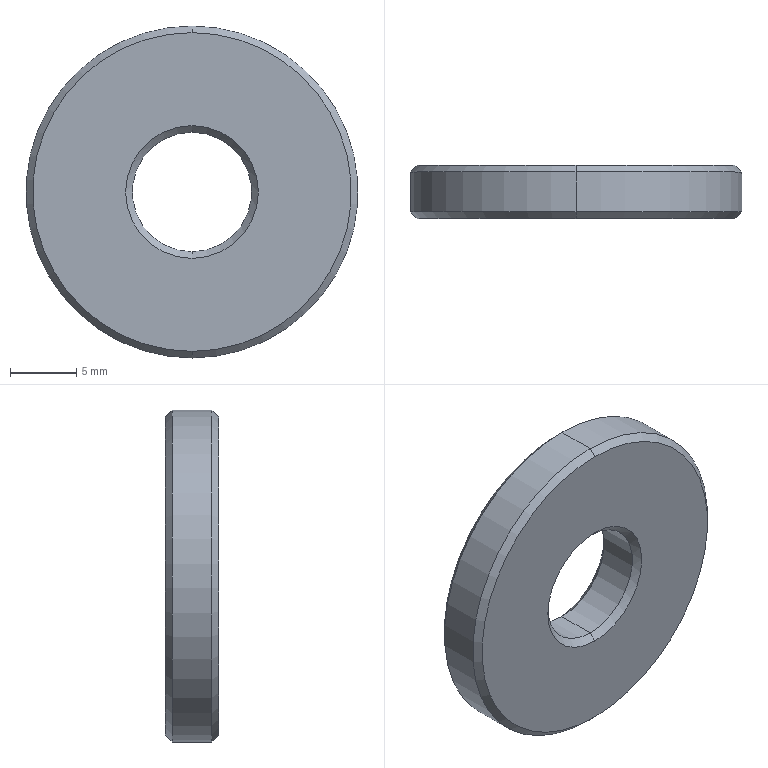Component | SolidWorks | Yk1.5.5EndCap-4 | 1 solid | 14 faces | box 25 x 4 x 25 mm | volume 1682 mm3 | cone 8 | cylinder 4 | plane 2 | commonest cylinder face diameters 9 x2 25 x2 | material 45
build123d program:
from build123d import *

# Parameters (mm, degrees)
SKETCH1_R           = 12.5
SKETCH1_R_2         = 4.5
BOSS_EXTRUDE1_DEPTH = 4
CHAMFER1_SIZE       = 0.5


with BuildPart() as part:
    # Sketch1 → Boss-Extrude1 (new body)
    with BuildSketch(Plane(origin=(0, 0, 0), x_dir=(1, 0, 0), z_dir=(0, 1, 0))):
        with Locations(Location((0, 0, 0), (0, 0, 270))):
            Circle(SKETCH1_R)
        with Locations(Location((0, 0, 0), (0, 0, 270))):
            Circle(SKETCH1_R_2, mode=Mode.SUBTRACT)
    extrude(amount=BOSS_EXTRUDE1_DEPTH)

    # Chamfer1
    chamfer1_edges = [part.edges().sort_by_distance(p)[0] for p in [
        (0, 0, -12.5),
        (0, 4, -12.5),
        (0, 0, -4.5),
        (0, 4, -4.5),
    ]]
    chamfer(chamfer1_edges, length=CHAMFER1_SIZE)


solid = part.part

# Placed as in the assembly
solid = solid.moved(Location((-41.072, -44, 23.739), (0, 0, 0)))
STEP:
#1=COLOUR_RGB('',0.7922,0.8196,0.9333);
#2=FILL_AREA_STYLE_COLOUR('',#1);
#3=FILL_AREA_STYLE('',(#2));
#4=SURFACE_STYLE_FILL_AREA(#3);
#5=SURFACE_SIDE_STYLE('',(#4));
#6=SURFACE_STYLE_USAGE(.BOTH.,#5);
#7=PRESENTATION_STYLE_ASSIGNMENT((#6));
#8=CARTESIAN_POINT('',(-1.617,-1.732,0.4621));
#9=VERTEX_POINT('',#8);
#10=CARTESIAN_POINT('',(-1.617,-1.732,1.407));
#11=VERTEX_POINT('',#10);
#12=CARTESIAN_POINT('',(-1.617,-1.732,0.9346));
#13=DIRECTION('',(0.,-1.,0.));
#14=DIRECTION('',(0.,0.,1.));
#15=AXIS2_PLACEMENT_3D('',#12,#13,#14);
#16=CIRCLE('',#15,0.4724);
#17=EDGE_CURVE('',#9,#11,#16,.T.);
#18=ORIENTED_EDGE('',*,*,#17,.F.);
#19=CARTESIAN_POINT('',(-1.617,-1.713,0.4425));
#20=VERTEX_POINT('',#19);
#21=CARTESIAN_POINT('',(-1.617,-1.713,0.4425));
#22=DIRECTION('',(0.,0.7071,-0.7071));
#23=VECTOR('',#22,39.37);
#24=LINE('',#21,#23);
#25=EDGE_CURVE('',#9,#20,#24,.T.);
#26=ORIENTED_EDGE('',*,*,#25,.T.);
#27=CARTESIAN_POINT('',(-1.617,-1.713,1.427));
#28=VERTEX_POINT('',#27);
#29=CARTESIAN_POINT('',(-1.617,-1.713,0.9346));
#30=DIRECTION('',(0.,1.,0.));
#31=DIRECTION('',(0.,0.,1.));
#32=AXIS2_PLACEMENT_3D('',#29,#30,#31);
#33=CIRCLE('',#32,0.4921);
#34=EDGE_CURVE('',#28,#20,#33,.T.);
#35=ORIENTED_EDGE('',*,*,#34,.F.);
#36=CARTESIAN_POINT('',(-1.617,-1.713,1.427));
#37=DIRECTION('',(0.,0.7071,0.7071));
#38=VECTOR('',#37,39.37);
#39=LINE('',#36,#38);
#40=EDGE_CURVE('',#11,#28,#39,.T.);
#41=ORIENTED_EDGE('',*,*,#40,.F.);
#42=EDGE_LOOP('',(#18,#26,#35,#41));
#43=FACE_OUTER_BOUND('',#42,.T.);
#44=CARTESIAN_POINT('',(-1.617,-1.713,0.9346));
#45=DIRECTION('',(0.,1.,0.));
#46=DIRECTION('',(0.,0.,1.));
#47=AXIS2_PLACEMENT_3D('',#44,#45,#46);
#48=CONICAL_SURFACE('',#47,0.4921,0.7854);
#49=ADVANCED_FACE('',(#43),#48,.T.);
#50=CARTESIAN_POINT('',(-1.617,-1.713,1.112));
#51=VERTEX_POINT('',#50);
#52=CARTESIAN_POINT('',(-1.617,-1.713,0.7574));
#53=VERTEX_POINT('',#52);
#54=CARTESIAN_POINT('',(-1.617,-1.713,0.9346));
#55=DIRECTION('',(0.,-1.,0.));
#56=DIRECTION('',(0.,0.,1.));
#57=AXIS2_PLACEMENT_3D('',#54,#55,#56);
#58=CIRCLE('',#57,0.1772);
#59=EDGE_CURVE('',#51,#53,#58,.T.);
#60=ORIENTED_EDGE('',*,*,#59,.F.);
#61=CARTESIAN_POINT('',(-1.617,-1.732,1.131));
#62=VERTEX_POINT('',#61);
#63=CARTESIAN_POINT('',(-1.617,-1.732,1.131));
#64=DIRECTION('',(0.,-0.7071,0.7071));
#65=VECTOR('',#64,39.37);
#66=LINE('',#63,#65);
#67=EDGE_CURVE('',#51,#62,#66,.T.);
#68=ORIENTED_EDGE('',*,*,#67,.T.);
#69=CARTESIAN_POINT('',(-1.617,-1.732,0.7377));
#70=VERTEX_POINT('',#69);
#71=CARTESIAN_POINT('',(-1.617,-1.732,0.9346));
#72=DIRECTION('',(0.,1.,0.));
#73=DIRECTION('',(0.,0.,1.));
#74=AXIS2_PLACEMENT_3D('',#71,#72,#73);
#75=CIRCLE('',#74,0.1969);
#76=EDGE_CURVE('',#70,#62,#75,.T.);
#77=ORIENTED_EDGE('',*,*,#76,.F.);
#78=CARTESIAN_POINT('',(-1.617,-1.732,0.7377));
#79=DIRECTION('',(0.,-0.7071,-0.7071));
#80=VECTOR('',#79,39.37);
#81=LINE('',#78,#80);
#82=EDGE_CURVE('',#53,#70,#81,.T.);
#83=ORIENTED_EDGE('',*,*,#82,.F.);
#84=EDGE_LOOP('',(#60,#68,#77,#83));
#85=FACE_OUTER_BOUND('',#84,.T.);
#86=CARTESIAN_POINT('',(-1.617,-1.732,0.9346));
#87=DIRECTION('',(0.,-1.,0.));
#88=DIRECTION('',(0.,0.,-1.));
#89=AXIS2_PLACEMENT_3D('',#86,#87,#88);
#90=CONICAL_SURFACE('',#89,0.1969,0.7854);
#91=ADVANCED_FACE('',(#85),#90,.F.);
#92=CARTESIAN_POINT('',(-1.617,-1.575,1.407));
#93=VERTEX_POINT('',#92);
#94=CARTESIAN_POINT('',(-1.617,-1.575,0.4621));
#95=VERTEX_POINT('',#94);
#96=CARTESIAN_POINT('',(-1.617,-1.575,0.9346));
#97=DIRECTION('',(0.,1.,0.));
#98=DIRECTION('',(0.,0.,1.));
#99=AXIS2_PLACEMENT_3D('',#96,#97,#98);
#100=CIRCLE('',#99,0.4724);
#101=EDGE_CURVE('',#93,#95,#100,.T.);
#102=ORIENTED_EDGE('',*,*,#101,.F.);
#103=CARTESIAN_POINT('',(-1.617,-1.594,1.427));
#104=VERTEX_POINT('',#103);
#105=CARTESIAN_POINT('',(-1.617,-1.575,1.407));
#106=DIRECTION('',(0.,-0.7071,0.7071));
#107=VECTOR('',#106,39.37);
#108=LINE('',#105,#107);
#109=EDGE_CURVE('',#93,#104,#108,.T.);
#110=ORIENTED_EDGE('',*,*,#109,.T.);
#111=CARTESIAN_POINT('',(-1.617,-1.594,0.4425));
#112=VERTEX_POINT('',#111);
#113=CARTESIAN_POINT('',(-1.617,-1.594,0.9346));
#114=DIRECTION('',(0.,-1.,0.));
#115=DIRECTION('',(0.,0.,1.));
#116=AXIS2_PLACEMENT_3D('',#113,#114,#115);
#117=CIRCLE('',#116,0.4921);
#118=EDGE_CURVE('',#112,#104,#117,.T.);
#119=ORIENTED_EDGE('',*,*,#118,.F.);
#120=CARTESIAN_POINT('',(-1.617,-1.575,0.4621));
#121=DIRECTION('',(0.,-0.7071,-0.7071));
#122=VECTOR('',#121,39.37);
#123=LINE('',#120,#122);
#124=EDGE_CURVE('',#95,#112,#123,.T.);
#125=ORIENTED_EDGE('',*,*,#124,.F.);
#126=EDGE_LOOP('',(#102,#110,#119,#125));
#127=FACE_OUTER_BOUND('',#126,.T.);
#128=CARTESIAN_POINT('',(-1.617,-1.575,0.9346));
#129=DIRECTION('',(0.,-1.,0.));
#130=DIRECTION('',(0.,0.,-1.));
#131=AXIS2_PLACEMENT_3D('',#128,#129,#130);
#132=CONICAL_SURFACE('',#131,0.4724,0.7854);
#133=ADVANCED_FACE('',(#127),#132,.T.);
#134=CARTESIAN_POINT('',(-1.617,-1.594,0.7574));
#135=VERTEX_POINT('',#134);
#136=CARTESIAN_POINT('',(-1.617,-1.594,1.112));
#137=VERTEX_POINT('',#136);
#138=CARTESIAN_POINT('',(-1.617,-1.594,0.9346));
#139=DIRECTION('',(0.,1.,0.));
#140=DIRECTION('',(0.,0.,1.));
#141=AXIS2_PLACEMENT_3D('',#138,#139,#140);
#142=CIRCLE('',#141,0.1772);
#143=EDGE_CURVE('',#135,#137,#142,.T.);
#144=ORIENTED_EDGE('',*,*,#143,.F.);
#145=CARTESIAN_POINT('',(-1.617,-1.575,0.7377));
#146=VERTEX_POINT('',#145);
#147=CARTESIAN_POINT('',(-1.617,-1.594,0.7574));
#148=DIRECTION('',(0.,0.7071,-0.7071));
#149=VECTOR('',#148,39.37);
#150=LINE('',#147,#149);
#151=EDGE_CURVE('',#135,#146,#150,.T.);
#152=ORIENTED_EDGE('',*,*,#151,.T.);
#153=CARTESIAN_POINT('',(-1.617,-1.575,1.131));
#154=VERTEX_POINT('',#153);
#155=CARTESIAN_POINT('',(-1.617,-1.575,0.9346));
#156=DIRECTION('',(0.,-1.,0.));
#157=DIRECTION('',(0.,0.,1.));
#158=AXIS2_PLACEMENT_3D('',#155,#156,#157);
#159=CIRCLE('',#158,0.1969);
#160=EDGE_CURVE('',#154,#146,#159,.T.);
#161=ORIENTED_EDGE('',*,*,#160,.F.);
#162=CARTESIAN_POINT('',(-1.617,-1.594,1.112));
#163=DIRECTION('',(0.,0.7071,0.7071));
#164=VECTOR('',#163,39.37);
#165=LINE('',#162,#164);
#166=EDGE_CURVE('',#137,#154,#165,.T.);
#167=ORIENTED_EDGE('',*,*,#166,.F.);
#168=EDGE_LOOP('',(#144,#152,#161,#167));
#169=FACE_OUTER_BOUND('',#168,.T.);
#170=CARTESIAN_POINT('',(-1.617,-1.594,0.9346));
#171=DIRECTION('',(0.,1.,0.));
#172=DIRECTION('',(0.,0.,1.));
#173=AXIS2_PLACEMENT_3D('',#170,#171,#172);
#174=CONICAL_SURFACE('',#173,0.1772,0.7854);
#175=ADVANCED_FACE('',(#169),#174,.F.);
#176=ORIENTED_EDGE('',*,*,#143,.T.);
#177=CARTESIAN_POINT('',(-1.617,-1.575,1.112));
#178=DIRECTION('',(0.,-1.,0.));
#179=VECTOR('',#178,39.37);
#180=LINE('',#177,#179);
#181=EDGE_CURVE('',#137,#51,#180,.T.);
#182=ORIENTED_EDGE('',*,*,#181,.T.);
#183=ORIENTED_EDGE('',*,*,#59,.T.);
#184=CARTESIAN_POINT('',(-1.617,-1.575,0.7574));
#185=DIRECTION('',(0.,-1.,0.));
#186=VECTOR('',#185,39.37);
#187=LINE('',#184,#186);
#188=EDGE_CURVE('',#135,#53,#187,.T.);
#189=ORIENTED_EDGE('',*,*,#188,.F.);
#190=EDGE_LOOP('',(#176,#182,#183,#189));
#191=FACE_OUTER_BOUND('',#190,.T.);
#192=CARTESIAN_POINT('',(-1.617,-1.575,0.9346));
#193=DIRECTION('',(0.,-1.,0.));
#194=DIRECTION('',(0.,0.,-1.));
#195=AXIS2_PLACEMENT_3D('',#192,#193,#194);
#196=CYLINDRICAL_SURFACE('',#195,0.1772);
#197=ADVANCED_FACE('',(#191),#196,.F.);
#198=ORIENTED_EDGE('',*,*,#118,.T.);
#199=CARTESIAN_POINT('',(-1.617,-1.575,1.427));
#200=DIRECTION('',(0.,-1.,0.));
#201=VECTOR('',#200,39.37);
#202=LINE('',#199,#201);
#203=EDGE_CURVE('',#104,#28,#202,.T.);
#204=ORIENTED_EDGE('',*,*,#203,.T.);
#205=ORIENTED_EDGE('',*,*,#34,.T.);
#206=CARTESIAN_POINT('',(-1.617,-1.575,0.4425));
#207=DIRECTION('',(0.,-1.,0.));
#208=VECTOR('',#207,39.37);
#209=LINE('',#206,#208);
#210=EDGE_CURVE('',#112,#20,#209,.T.);
#211=ORIENTED_EDGE('',*,*,#210,.F.);
#212=EDGE_LOOP('',(#198,#204,#205,#211));
#213=FACE_OUTER_BOUND('',#212,.T.);
#214=CARTESIAN_POINT('',(-1.617,-1.575,0.9346));
#215=DIRECTION('',(0.,-1.,0.));
#216=DIRECTION('',(0.,0.,-1.));
#217=AXIS2_PLACEMENT_3D('',#214,#215,#216);
#218=CYLINDRICAL_SURFACE('',#217,0.4921);
#219=ADVANCED_FACE('',(#213),#218,.T.);
#220=ORIENTED_EDGE('',*,*,#160,.T.);
#221=CARTESIAN_POINT('',(-1.617,-1.575,0.9346));
#222=DIRECTION('',(0.,-1.,0.));
#223=DIRECTION('',(0.,0.,1.));
#224=AXIS2_PLACEMENT_3D('',#221,#222,#223);
#225=CIRCLE('',#224,0.1969);
#226=EDGE_CURVE('',#146,#154,#225,.T.);
#227=ORIENTED_EDGE('',*,*,#226,.T.);
#228=EDGE_LOOP('',(#220,#227));
#229=FACE_BOUND('',#228,.T.);
#230=CARTESIAN_POINT('',(-1.617,-1.575,0.9346));
#231=DIRECTION('',(0.,1.,0.));
#232=DIRECTION('',(0.,0.,1.));
#233=AXIS2_PLACEMENT_3D('',#230,#231,#232);
#234=CIRCLE('',#233,0.4724);
#235=EDGE_CURVE('',#95,#93,#234,.T.);
#236=ORIENTED_EDGE('',*,*,#235,.T.);
#237=ORIENTED_EDGE('',*,*,#101,.T.);
#238=EDGE_LOOP('',(#236,#237));
#239=FACE_OUTER_BOUND('',#238,.T.);
#240=CARTESIAN_POINT('',(-1.617,-1.575,0.9346));
#241=DIRECTION('',(0.,1.,0.));
#242=DIRECTION('',(0.,0.,1.));
#243=AXIS2_PLACEMENT_3D('',#240,#241,#242);
#244=PLANE('',#243);
#245=ADVANCED_FACE('',(#229,#239),#244,.T.);
#246=ORIENTED_EDGE('',*,*,#76,.T.);
#247=CARTESIAN_POINT('',(-1.617,-1.732,0.9346));
#248=DIRECTION('',(0.,1.,0.));
#249=DIRECTION('',(0.,0.,1.));
#250=AXIS2_PLACEMENT_3D('',#247,#248,#249);
#251=CIRCLE('',#250,0.1969);
#252=EDGE_CURVE('',#62,#70,#251,.T.);
#253=ORIENTED_EDGE('',*,*,#252,.T.);
#254=EDGE_LOOP('',(#246,#253));
#255=FACE_BOUND('',#254,.T.);
#256=CARTESIAN_POINT('',(-1.617,-1.732,0.9346));
#257=DIRECTION('',(0.,-1.,0.));
#258=DIRECTION('',(0.,0.,1.));
#259=AXIS2_PLACEMENT_3D('',#256,#257,#258);
#260=CIRCLE('',#259,0.4724);
#261=EDGE_CURVE('',#11,#9,#260,.T.);
#262=ORIENTED_EDGE('',*,*,#261,.T.);
#263=ORIENTED_EDGE('',*,*,#17,.T.);
#264=EDGE_LOOP('',(#262,#263));
#265=FACE_OUTER_BOUND('',#264,.T.);
#266=CARTESIAN_POINT('',(-1.617,-1.732,0.9346));
#267=DIRECTION('',(0.,1.,0.));
#268=DIRECTION('',(0.,0.,1.));
#269=AXIS2_PLACEMENT_3D('',#266,#267,#268);
#270=PLANE('',#269);
#271=ADVANCED_FACE('',(#255,#265),#270,.F.);
#272=ORIENTED_EDGE('',*,*,#203,.F.);
#273=CARTESIAN_POINT('',(-1.617,-1.594,0.9346));
#274=DIRECTION('',(0.,-1.,0.));
#275=DIRECTION('',(0.,0.,1.));
#276=AXIS2_PLACEMENT_3D('',#273,#274,#275);
#277=CIRCLE('',#276,0.4921);
#278=EDGE_CURVE('',#104,#112,#277,.T.);
#279=ORIENTED_EDGE('',*,*,#278,.T.);
#280=ORIENTED_EDGE('',*,*,#210,.T.);
#281=CARTESIAN_POINT('',(-1.617,-1.713,0.9346));
#282=DIRECTION('',(0.,1.,0.));
#283=DIRECTION('',(0.,0.,1.));
#284=AXIS2_PLACEMENT_3D('',#281,#282,#283);
#285=CIRCLE('',#284,0.4921);
#286=EDGE_CURVE('',#20,#28,#285,.T.);
#287=ORIENTED_EDGE('',*,*,#286,.T.);
#288=EDGE_LOOP('',(#272,#279,#280,#287));
#289=FACE_OUTER_BOUND('',#288,.T.);
#290=CARTESIAN_POINT('',(-1.617,-1.575,0.9346));
#291=DIRECTION('',(0.,-1.,0.));
#292=DIRECTION('',(0.,0.,-1.));
#293=AXIS2_PLACEMENT_3D('',#290,#291,#292);
#294=CYLINDRICAL_SURFACE('',#293,0.4921);
#295=ADVANCED_FACE('',(#289),#294,.T.);
#296=ORIENTED_EDGE('',*,*,#181,.F.);
#297=CARTESIAN_POINT('',(-1.617,-1.594,0.9346));
#298=DIRECTION('',(0.,1.,0.));
#299=DIRECTION('',(0.,0.,1.));
#300=AXIS2_PLACEMENT_3D('',#297,#298,#299);
#301=CIRCLE('',#300,0.1772);
#302=EDGE_CURVE('',#137,#135,#301,.T.);
#303=ORIENTED_EDGE('',*,*,#302,.T.);
#304=ORIENTED_EDGE('',*,*,#188,.T.);
#305=CARTESIAN_POINT('',(-1.617,-1.713,0.9346));
#306=DIRECTION('',(0.,-1.,0.));
#307=DIRECTION('',(0.,0.,1.));
#308=AXIS2_PLACEMENT_3D('',#305,#306,#307);
#309=CIRCLE('',#308,0.1772);
#310=EDGE_CURVE('',#53,#51,#309,.T.);
#311=ORIENTED_EDGE('',*,*,#310,.T.);
#312=EDGE_LOOP('',(#296,#303,#304,#311));
#313=FACE_OUTER_BOUND('',#312,.T.);
#314=CARTESIAN_POINT('',(-1.617,-1.575,0.9346));
#315=DIRECTION('',(0.,-1.,0.));
#316=DIRECTION('',(0.,0.,-1.));
#317=AXIS2_PLACEMENT_3D('',#314,#315,#316);
#318=CYLINDRICAL_SURFACE('',#317,0.1772);
#319=ADVANCED_FACE('',(#313),#318,.F.);
#320=ORIENTED_EDGE('',*,*,#151,.F.);
#321=ORIENTED_EDGE('',*,*,#302,.F.);
#322=ORIENTED_EDGE('',*,*,#166,.T.);
#323=ORIENTED_EDGE('',*,*,#226,.F.);
#324=EDGE_LOOP('',(#320,#321,#322,#323));
#325=FACE_OUTER_BOUND('',#324,.T.);
#326=CARTESIAN_POINT('',(-1.617,-1.594,0.9346));
#327=DIRECTION('',(0.,1.,0.));
#328=DIRECTION('',(0.,0.,1.));
#329=AXIS2_PLACEMENT_3D('',#326,#327,#328);
#330=CONICAL_SURFACE('',#329,0.1772,0.7854);
#331=ADVANCED_FACE('',(#325),#330,.F.);
#332=ORIENTED_EDGE('',*,*,#109,.F.);
#333=ORIENTED_EDGE('',*,*,#235,.F.);
#334=ORIENTED_EDGE('',*,*,#124,.T.);
#335=ORIENTED_EDGE('',*,*,#278,.F.);
#336=EDGE_LOOP('',(#332,#333,#334,#335));
#337=FACE_OUTER_BOUND('',#336,.T.);
#338=CARTESIAN_POINT('',(-1.617,-1.575,0.9346));
#339=DIRECTION('',(0.,-1.,0.));
#340=DIRECTION('',(0.,0.,-1.));
#341=AXIS2_PLACEMENT_3D('',#338,#339,#340);
#342=CONICAL_SURFACE('',#341,0.4724,0.7854);
#343=ADVANCED_FACE('',(#337),#342,.T.);
#344=ORIENTED_EDGE('',*,*,#67,.F.);
#345=ORIENTED_EDGE('',*,*,#310,.F.);
#346=ORIENTED_EDGE('',*,*,#82,.T.);
#347=ORIENTED_EDGE('',*,*,#252,.F.);
#348=EDGE_LOOP('',(#344,#345,#346,#347));
#349=FACE_OUTER_BOUND('',#348,.T.);
#350=CARTESIAN_POINT('',(-1.617,-1.732,0.9346));
#351=DIRECTION('',(0.,-1.,0.));
#352=DIRECTION('',(0.,0.,-1.));
#353=AXIS2_PLACEMENT_3D('',#350,#351,#352);
#354=CONICAL_SURFACE('',#353,0.1969,0.7854);
#355=ADVANCED_FACE('',(#349),#354,.F.);
#356=ORIENTED_EDGE('',*,*,#25,.F.);
#357=ORIENTED_EDGE('',*,*,#261,.F.);
#358=ORIENTED_EDGE('',*,*,#40,.T.);
#359=ORIENTED_EDGE('',*,*,#286,.F.);
#360=EDGE_LOOP('',(#356,#357,#358,#359));
#361=FACE_OUTER_BOUND('',#360,.T.);
#362=CARTESIAN_POINT('',(-1.617,-1.713,0.9346));
#363=DIRECTION('',(0.,1.,0.));
#364=DIRECTION('',(0.,0.,1.));
#365=AXIS2_PLACEMENT_3D('',#362,#363,#364);
#366=CONICAL_SURFACE('',#365,0.4921,0.7854);
#367=ADVANCED_FACE('',(#361),#366,.T.);
#368=CLOSED_SHELL('',(#49,#91,#133,#175,#197,#219,#245,#271,#295,#319,#331,#343,#355,#367));
#369=MANIFOLD_SOLID_BREP('',#368);
#370=STYLED_ITEM('',(#7),#369);
#371=(LENGTH_UNIT()NAMED_UNIT(*)SI_UNIT($,.METRE.));
#372=LENGTH_MEASURE_WITH_UNIT(LENGTH_MEASURE(0.0254),#371);
#373=DIMENSIONAL_EXPONENTS(1.,0.,0.,0.,0.,0.,0.);
#374=(CONVERSION_BASED_UNIT('',#372)LENGTH_UNIT()NAMED_UNIT(#373));
#375=UNCERTAINTY_MEASURE_WITH_UNIT(LENGTH_MEASURE(0.00001),#374,'','');
#376=(NAMED_UNIT(*)PLANE_ANGLE_UNIT()SI_UNIT($,.RADIAN.));
#377=(NAMED_UNIT(*)SI_UNIT($,.STERADIAN.)SOLID_ANGLE_UNIT());
#378=(GEOMETRIC_REPRESENTATION_CONTEXT(3)GLOBAL_UNCERTAINTY_ASSIGNED_CONTEXT((#375))GLOBAL_UNIT_ASSIGNED_CONTEXT((#374,#376,#377))REPRESENTATION_CONTEXT('',''));
#379=MECHANICAL_DESIGN_GEOMETRIC_PRESENTATION_REPRESENTATION('',(#370),#378);
#380=PRESENTATION_LAYER_ASSIGNMENT('','',(#370));
#381=CARTESIAN_POINT('',(0.,0.,0.));
#382=DIRECTION('',(0.,0.,1.));
#383=DIRECTION('',(1.,0.,0.));
#384=AXIS2_PLACEMENT_3D('',#381,#382,#383);
#385=(LENGTH_UNIT()NAMED_UNIT(*)SI_UNIT($,.METRE.));
#386=LENGTH_MEASURE_WITH_UNIT(LENGTH_MEASURE(0.0254),#385);
#387=DIMENSIONAL_EXPONENTS(1.,0.,0.,0.,0.,0.,0.);
#388=(CONVERSION_BASED_UNIT('',#386)LENGTH_UNIT()NAMED_UNIT(#387));
#389=UNCERTAINTY_MEASURE_WITH_UNIT(LENGTH_MEASURE(0.00001),#388,'','');
#390=(NAMED_UNIT(*)PLANE_ANGLE_UNIT()SI_UNIT($,.RADIAN.));
#391=(NAMED_UNIT(*)SI_UNIT($,.STERADIAN.)SOLID_ANGLE_UNIT());
#392=(GEOMETRIC_REPRESENTATION_CONTEXT(3)GLOBAL_UNCERTAINTY_ASSIGNED_CONTEXT((#389))GLOBAL_UNIT_ASSIGNED_CONTEXT((#388,#390,#391))REPRESENTATION_CONTEXT('',''));
#393=ADVANCED_BREP_SHAPE_REPRESENTATION('',(#369,#384),#392);